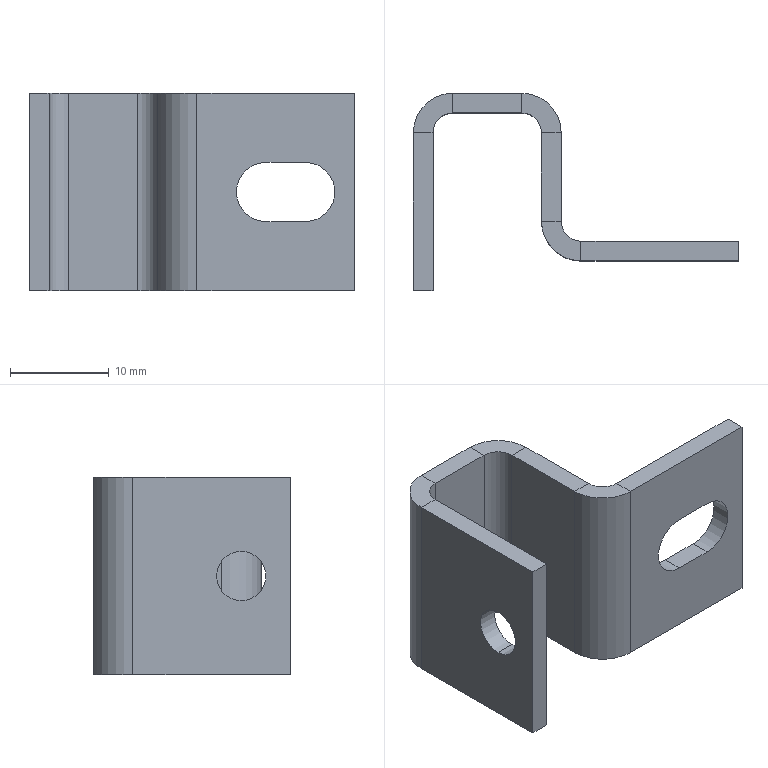Component | SolidWorks | Bracket(Item51)-1 | 1 solid | 36 faces | box 33 x 20 x 20 mm | volume 2342 mm3 | plane 26 | cylinder 10 | commonest cylinder face diameters 8 x3 4 x3 5 x2 6 x2 | material Plain Carbon Steel
STEP:
#1=COLOUR_RGB('',0.7922,0.8196,0.9333);
#2=FILL_AREA_STYLE_COLOUR('',#1);
#3=FILL_AREA_STYLE('',(#2));
#4=SURFACE_STYLE_FILL_AREA(#3);
#5=SURFACE_SIDE_STYLE('',(#4));
#6=SURFACE_STYLE_USAGE(.BOTH.,#5);
#7=PRESENTATION_STYLE_ASSIGNMENT((#6));
#8=CARTESIAN_POINT('',(-16.26,14.764,-4.528));
#9=VERTEX_POINT('',#8);
#10=CARTESIAN_POINT('',(-16.26,14.764,-4.331));
#11=VERTEX_POINT('',#10);
#12=CARTESIAN_POINT('',(-16.26,14.764,-4.429));
#13=DIRECTION('',(1.,-0.,0.));
#14=DIRECTION('',(0.,-1.,0.));
#15=AXIS2_PLACEMENT_3D('',#12,#13,#14);
#16=CIRCLE('',#15,0.09843);
#17=EDGE_CURVE('',#9,#11,#16,.T.);
#18=ORIENTED_EDGE('',*,*,#17,.T.);
#19=CARTESIAN_POINT('',(-16.339,14.764,-4.331));
#20=VERTEX_POINT('',#19);
#21=CARTESIAN_POINT('',(-16.339,14.764,-4.331));
#22=DIRECTION('',(-1.,0.,-0.));
#23=VECTOR('',#22,39.37);
#24=LINE('',#21,#23);
#25=EDGE_CURVE('',#11,#20,#24,.T.);
#26=ORIENTED_EDGE('',*,*,#25,.T.);
#27=CARTESIAN_POINT('',(-16.339,14.764,-4.528));
#28=VERTEX_POINT('',#27);
#29=CARTESIAN_POINT('',(-16.339,14.764,-4.429));
#30=DIRECTION('',(-1.,0.,-0.));
#31=DIRECTION('',(0.,0.,-1.));
#32=AXIS2_PLACEMENT_3D('',#29,#30,#31);
#33=CIRCLE('',#32,0.09843);
#34=EDGE_CURVE('',#20,#28,#33,.T.);
#35=ORIENTED_EDGE('',*,*,#34,.T.);
#36=CARTESIAN_POINT('',(-16.339,14.764,-4.528));
#37=DIRECTION('',(-1.,0.,-0.));
#38=VECTOR('',#37,39.37);
#39=LINE('',#36,#38);
#40=EDGE_CURVE('',#9,#28,#39,.T.);
#41=ORIENTED_EDGE('',*,*,#40,.F.);
#42=EDGE_LOOP('',(#18,#26,#35,#41));
#43=FACE_OUTER_BOUND('',#42,.T.);
#44=CARTESIAN_POINT('',(-16.339,14.764,-4.429));
#45=DIRECTION('',(-1.,0.,-0.));
#46=DIRECTION('',(0.,0.,-1.));
#47=AXIS2_PLACEMENT_3D('',#44,#45,#46);
#48=CYLINDRICAL_SURFACE('',#47,0.09843);
#49=ADVANCED_FACE('',(#43),#48,.F.);
#50=CARTESIAN_POINT('',(-16.339,15.197,-4.823));
#51=VERTEX_POINT('',#50);
#52=CARTESIAN_POINT('',(-16.26,15.197,-4.823));
#53=VERTEX_POINT('',#52);
#54=CARTESIAN_POINT('',(-16.339,15.197,-4.823));
#55=DIRECTION('',(1.,-0.,0.));
#56=VECTOR('',#55,39.37);
#57=LINE('',#54,#56);
#58=EDGE_CURVE('',#51,#53,#57,.T.);
#59=ORIENTED_EDGE('',*,*,#58,.F.);
#60=CARTESIAN_POINT('',(-16.181,15.354,-4.823));
#61=VERTEX_POINT('',#60);
#62=CARTESIAN_POINT('',(-16.181,15.197,-4.823));
#63=DIRECTION('',(0.,-0.,-1.));
#64=DIRECTION('',(-1.,0.,0.));
#65=AXIS2_PLACEMENT_3D('',#62,#63,#64);
#66=CIRCLE('',#65,0.1575);
#67=EDGE_CURVE('',#51,#61,#66,.T.);
#68=ORIENTED_EDGE('',*,*,#67,.T.);
#69=CARTESIAN_POINT('',(-16.181,15.276,-4.823));
#70=VERTEX_POINT('',#69);
#71=CARTESIAN_POINT('',(-16.181,15.276,-4.823));
#72=DIRECTION('',(0.,1.,-0.));
#73=VECTOR('',#72,39.37);
#74=LINE('',#71,#73);
#75=EDGE_CURVE('',#70,#61,#74,.T.);
#76=ORIENTED_EDGE('',*,*,#75,.F.);
#77=CARTESIAN_POINT('',(-16.181,15.197,-4.823));
#78=DIRECTION('',(0.,-0.,-1.));
#79=DIRECTION('',(1.,0.,0.));
#80=AXIS2_PLACEMENT_3D('',#77,#78,#79);
#81=CIRCLE('',#80,0.07874);
#82=EDGE_CURVE('',#53,#70,#81,.T.);
#83=ORIENTED_EDGE('',*,*,#82,.F.);
#84=EDGE_LOOP('',(#59,#68,#76,#83));
#85=FACE_OUTER_BOUND('',#84,.T.);
#86=CARTESIAN_POINT('',(-16.339,15.197,-4.823));
#87=DIRECTION('',(0.,-0.,-1.));
#88=DIRECTION('',(1.,-0.,0.));
#89=AXIS2_PLACEMENT_3D('',#86,#87,#88);
#90=PLANE('',#89);
#91=ADVANCED_FACE('',(#85),#90,.T.);
#92=CARTESIAN_POINT('',(-16.339,14.567,-4.823));
#93=VERTEX_POINT('',#92);
#94=CARTESIAN_POINT('',(-16.339,14.567,-4.823));
#95=DIRECTION('',(0.,1.,-0.));
#96=VECTOR('',#95,39.37);
#97=LINE('',#94,#96);
#98=EDGE_CURVE('',#93,#51,#97,.T.);
#99=ORIENTED_EDGE('',*,*,#98,.T.);
#100=ORIENTED_EDGE('',*,*,#58,.T.);
#101=CARTESIAN_POINT('',(-16.26,14.567,-4.823));
#102=VERTEX_POINT('',#101);
#103=CARTESIAN_POINT('',(-16.26,14.567,-4.823));
#104=DIRECTION('',(0.,1.,-0.));
#105=VECTOR('',#104,39.37);
#106=LINE('',#103,#105);
#107=EDGE_CURVE('',#102,#53,#106,.T.);
#108=ORIENTED_EDGE('',*,*,#107,.F.);
#109=CARTESIAN_POINT('',(-16.339,14.567,-4.823));
#110=DIRECTION('',(1.,-0.,0.));
#111=VECTOR('',#110,39.37);
#112=LINE('',#109,#111);
#113=EDGE_CURVE('',#93,#102,#112,.T.);
#114=ORIENTED_EDGE('',*,*,#113,.F.);
#115=EDGE_LOOP('',(#99,#100,#108,#114));
#116=FACE_OUTER_BOUND('',#115,.T.);
#117=CARTESIAN_POINT('',(-16.181,15.276,-4.823));
#118=DIRECTION('',(0.,-0.,-1.));
#119=DIRECTION('',(1.,-0.,0.));
#120=AXIS2_PLACEMENT_3D('',#117,#118,#119);
#121=PLANE('',#120);
#122=ADVANCED_FACE('',(#116),#121,.T.);
#123=CARTESIAN_POINT('',(-16.181,15.354,-4.035));
#124=VERTEX_POINT('',#123);
#125=CARTESIAN_POINT('',(-16.181,15.276,-4.035));
#126=VERTEX_POINT('',#125);
#127=CARTESIAN_POINT('',(-16.181,15.354,-4.035));
#128=DIRECTION('',(-0.,-1.,0.));
#129=VECTOR('',#128,39.37);
#130=LINE('',#127,#129);
#131=EDGE_CURVE('',#124,#126,#130,.T.);
#132=ORIENTED_EDGE('',*,*,#131,.F.);
#133=CARTESIAN_POINT('',(-16.339,15.197,-4.035));
#134=VERTEX_POINT('',#133);
#135=CARTESIAN_POINT('',(-16.181,15.197,-4.035));
#136=DIRECTION('',(0.,-0.,-1.));
#137=DIRECTION('',(-1.,0.,0.));
#138=AXIS2_PLACEMENT_3D('',#135,#136,#137);
#139=CIRCLE('',#138,0.1575);
#140=EDGE_CURVE('',#134,#124,#139,.T.);
#141=ORIENTED_EDGE('',*,*,#140,.F.);
#142=CARTESIAN_POINT('',(-16.26,15.197,-4.035));
#143=VERTEX_POINT('',#142);
#144=CARTESIAN_POINT('',(-16.26,15.197,-4.035));
#145=DIRECTION('',(-1.,0.,-0.));
#146=VECTOR('',#145,39.37);
#147=LINE('',#144,#146);
#148=EDGE_CURVE('',#143,#134,#147,.T.);
#149=ORIENTED_EDGE('',*,*,#148,.F.);
#150=CARTESIAN_POINT('',(-16.181,15.197,-4.035));
#151=DIRECTION('',(0.,-0.,-1.));
#152=DIRECTION('',(1.,0.,0.));
#153=AXIS2_PLACEMENT_3D('',#150,#151,#152);
#154=CIRCLE('',#153,0.07874);
#155=EDGE_CURVE('',#143,#126,#154,.T.);
#156=ORIENTED_EDGE('',*,*,#155,.T.);
#157=EDGE_LOOP('',(#132,#141,#149,#156));
#158=FACE_OUTER_BOUND('',#157,.T.);
#159=CARTESIAN_POINT('',(-16.181,15.354,-4.035));
#160=DIRECTION('',(-0.,0.,1.));
#161=DIRECTION('',(-1.,0.,-0.));
#162=AXIS2_PLACEMENT_3D('',#159,#160,#161);
#163=PLANE('',#162);
#164=ADVANCED_FACE('',(#158),#163,.T.);
#165=CARTESIAN_POINT('',(-15.906,15.354,-4.035));
#166=VERTEX_POINT('',#165);
#167=CARTESIAN_POINT('',(-16.339,15.354,-4.035));
#168=DIRECTION('',(1.,-0.,0.));
#169=VECTOR('',#168,39.37);
#170=LINE('',#167,#169);
#171=EDGE_CURVE('',#124,#166,#170,.T.);
#172=ORIENTED_EDGE('',*,*,#171,.F.);
#173=ORIENTED_EDGE('',*,*,#131,.T.);
#174=CARTESIAN_POINT('',(-15.906,15.276,-4.035));
#175=VERTEX_POINT('',#174);
#176=CARTESIAN_POINT('',(-16.339,15.276,-4.035));
#177=DIRECTION('',(1.,-0.,0.));
#178=VECTOR('',#177,39.37);
#179=LINE('',#176,#178);
#180=EDGE_CURVE('',#126,#175,#179,.T.);
#181=ORIENTED_EDGE('',*,*,#180,.T.);
#182=CARTESIAN_POINT('',(-15.906,15.276,-4.035));
#183=DIRECTION('',(-0.,1.,-0.));
#184=VECTOR('',#183,39.37);
#185=LINE('',#182,#184);
#186=EDGE_CURVE('',#175,#166,#185,.T.);
#187=ORIENTED_EDGE('',*,*,#186,.T.);
#188=EDGE_LOOP('',(#172,#173,#181,#187));
#189=FACE_OUTER_BOUND('',#188,.T.);
#190=CARTESIAN_POINT('',(-16.26,15.197,-4.035));
#191=DIRECTION('',(-0.,0.,1.));
#192=DIRECTION('',(-1.,0.,-0.));
#193=AXIS2_PLACEMENT_3D('',#190,#191,#192);
#194=PLANE('',#193);
#195=ADVANCED_FACE('',(#189),#194,.T.);
#196=CARTESIAN_POINT('',(-15.906,15.354,-4.823));
#197=VERTEX_POINT('',#196);
#198=CARTESIAN_POINT('',(-15.906,15.276,-4.823));
#199=VERTEX_POINT('',#198);
#200=CARTESIAN_POINT('',(-15.906,15.354,-4.823));
#201=DIRECTION('',(0.,-1.,0.));
#202=VECTOR('',#201,39.37);
#203=LINE('',#200,#202);
#204=EDGE_CURVE('',#197,#199,#203,.T.);
#205=ORIENTED_EDGE('',*,*,#204,.F.);
#206=CARTESIAN_POINT('',(-15.748,15.197,-4.823));
#207=VERTEX_POINT('',#206);
#208=CARTESIAN_POINT('',(-15.906,15.197,-4.823));
#209=DIRECTION('',(0.,-0.,-1.));
#210=DIRECTION('',(-1.,0.,0.));
#211=AXIS2_PLACEMENT_3D('',#208,#209,#210);
#212=CIRCLE('',#211,0.1575);
#213=EDGE_CURVE('',#197,#207,#212,.T.);
#214=ORIENTED_EDGE('',*,*,#213,.T.);
#215=CARTESIAN_POINT('',(-15.827,15.197,-4.823));
#216=VERTEX_POINT('',#215);
#217=CARTESIAN_POINT('',(-15.827,15.197,-4.823));
#218=DIRECTION('',(1.,-0.,0.));
#219=VECTOR('',#218,39.37);
#220=LINE('',#217,#219);
#221=EDGE_CURVE('',#216,#207,#220,.T.);
#222=ORIENTED_EDGE('',*,*,#221,.F.);
#223=CARTESIAN_POINT('',(-15.906,15.197,-4.823));
#224=DIRECTION('',(0.,-0.,-1.));
#225=DIRECTION('',(1.,0.,0.));
#226=AXIS2_PLACEMENT_3D('',#223,#224,#225);
#227=CIRCLE('',#226,0.07874);
#228=EDGE_CURVE('',#199,#216,#227,.T.);
#229=ORIENTED_EDGE('',*,*,#228,.F.);
#230=EDGE_LOOP('',(#205,#214,#222,#229));
#231=FACE_OUTER_BOUND('',#230,.T.);
#232=CARTESIAN_POINT('',(-15.906,15.354,-4.823));
#233=DIRECTION('',(0.,-0.,-1.));
#234=DIRECTION('',(1.,-0.,0.));
#235=AXIS2_PLACEMENT_3D('',#232,#233,#234);
#236=PLANE('',#235);
#237=ADVANCED_FACE('',(#231),#236,.T.);
#238=CARTESIAN_POINT('',(-16.339,15.354,-4.823));
#239=DIRECTION('',(1.,-0.,0.));
#240=VECTOR('',#239,39.37);
#241=LINE('',#238,#240);
#242=EDGE_CURVE('',#61,#197,#241,.T.);
#243=ORIENTED_EDGE('',*,*,#242,.T.);
#244=ORIENTED_EDGE('',*,*,#204,.T.);
#245=CARTESIAN_POINT('',(-16.339,15.276,-4.823));
#246=DIRECTION('',(1.,-0.,0.));
#247=VECTOR('',#246,39.37);
#248=LINE('',#245,#247);
#249=EDGE_CURVE('',#70,#199,#248,.T.);
#250=ORIENTED_EDGE('',*,*,#249,.F.);
#251=ORIENTED_EDGE('',*,*,#75,.T.);
#252=EDGE_LOOP('',(#243,#244,#250,#251));
#253=FACE_OUTER_BOUND('',#252,.T.);
#254=CARTESIAN_POINT('',(-15.827,15.197,-4.823));
#255=DIRECTION('',(0.,-0.,-1.));
#256=DIRECTION('',(1.,-0.,0.));
#257=AXIS2_PLACEMENT_3D('',#254,#255,#256);
#258=PLANE('',#257);
#259=ADVANCED_FACE('',(#253),#258,.T.);
#260=CARTESIAN_POINT('',(-15.748,15.197,-4.035));
#261=VERTEX_POINT('',#260);
#262=CARTESIAN_POINT('',(-15.827,15.197,-4.035));
#263=VERTEX_POINT('',#262);
#264=CARTESIAN_POINT('',(-15.748,15.197,-4.035));
#265=DIRECTION('',(-1.,0.,-0.));
#266=VECTOR('',#265,39.37);
#267=LINE('',#264,#266);
#268=EDGE_CURVE('',#261,#263,#267,.T.);
#269=ORIENTED_EDGE('',*,*,#268,.F.);
#270=CARTESIAN_POINT('',(-15.906,15.197,-4.035));
#271=DIRECTION('',(0.,-0.,-1.));
#272=DIRECTION('',(-1.,0.,0.));
#273=AXIS2_PLACEMENT_3D('',#270,#271,#272);
#274=CIRCLE('',#273,0.1575);
#275=EDGE_CURVE('',#166,#261,#274,.T.);
#276=ORIENTED_EDGE('',*,*,#275,.F.);
#277=ORIENTED_EDGE('',*,*,#186,.F.);
#278=CARTESIAN_POINT('',(-15.906,15.197,-4.035));
#279=DIRECTION('',(0.,-0.,-1.));
#280=DIRECTION('',(1.,0.,0.));
#281=AXIS2_PLACEMENT_3D('',#278,#279,#280);
#282=CIRCLE('',#281,0.07874);
#283=EDGE_CURVE('',#175,#263,#282,.T.);
#284=ORIENTED_EDGE('',*,*,#283,.T.);
#285=EDGE_LOOP('',(#269,#276,#277,#284));
#286=FACE_OUTER_BOUND('',#285,.T.);
#287=CARTESIAN_POINT('',(-15.748,15.197,-4.035));
#288=DIRECTION('',(-0.,0.,1.));
#289=DIRECTION('',(-1.,0.,-0.));
#290=AXIS2_PLACEMENT_3D('',#287,#288,#289);
#291=PLANE('',#290);
#292=ADVANCED_FACE('',(#286),#291,.T.);
#293=CARTESIAN_POINT('',(-15.748,14.843,-4.035));
#294=VERTEX_POINT('',#293);
#295=CARTESIAN_POINT('',(-15.748,15.354,-4.035));
#296=DIRECTION('',(0.,-1.,0.));
#297=VECTOR('',#296,39.37);
#298=LINE('',#295,#297);
#299=EDGE_CURVE('',#261,#294,#298,.T.);
#300=ORIENTED_EDGE('',*,*,#299,.F.);
#301=ORIENTED_EDGE('',*,*,#268,.T.);
#302=CARTESIAN_POINT('',(-15.827,14.843,-4.035));
#303=VERTEX_POINT('',#302);
#304=CARTESIAN_POINT('',(-15.827,15.354,-4.035));
#305=DIRECTION('',(0.,-1.,0.));
#306=VECTOR('',#305,39.37);
#307=LINE('',#304,#306);
#308=EDGE_CURVE('',#263,#303,#307,.T.);
#309=ORIENTED_EDGE('',*,*,#308,.T.);
#310=CARTESIAN_POINT('',(-15.827,14.843,-4.035));
#311=DIRECTION('',(1.,0.,0.));
#312=VECTOR('',#311,39.37);
#313=LINE('',#310,#312);
#314=EDGE_CURVE('',#303,#294,#313,.T.);
#315=ORIENTED_EDGE('',*,*,#314,.T.);
#316=EDGE_LOOP('',(#300,#301,#309,#315));
#317=FACE_OUTER_BOUND('',#316,.T.);
#318=CARTESIAN_POINT('',(-15.906,15.276,-4.035));
#319=DIRECTION('',(-0.,0.,1.));
#320=DIRECTION('',(-1.,0.,-0.));
#321=AXIS2_PLACEMENT_3D('',#318,#319,#320);
#322=PLANE('',#321);
#323=ADVANCED_FACE('',(#317),#322,.T.);
#324=CARTESIAN_POINT('',(-15.748,14.843,-4.823));
#325=VERTEX_POINT('',#324);
#326=CARTESIAN_POINT('',(-15.827,14.843,-4.823));
#327=VERTEX_POINT('',#326);
#328=CARTESIAN_POINT('',(-15.748,14.843,-4.823));
#329=DIRECTION('',(-1.,-0.,-0.));
#330=VECTOR('',#329,39.37);
#331=LINE('',#328,#330);
#332=EDGE_CURVE('',#325,#327,#331,.T.);
#333=ORIENTED_EDGE('',*,*,#332,.F.);
#334=CARTESIAN_POINT('',(-15.669,14.764,-4.823));
#335=VERTEX_POINT('',#334);
#336=CARTESIAN_POINT('',(-15.669,14.843,-4.823));
#337=DIRECTION('',(-0.,0.,1.));
#338=DIRECTION('',(1.,0.,0.));
#339=AXIS2_PLACEMENT_3D('',#336,#337,#338);
#340=CIRCLE('',#339,0.07874);
#341=EDGE_CURVE('',#325,#335,#340,.T.);
#342=ORIENTED_EDGE('',*,*,#341,.T.);
#343=CARTESIAN_POINT('',(-15.669,14.685,-4.823));
#344=VERTEX_POINT('',#343);
#345=CARTESIAN_POINT('',(-15.669,14.685,-4.823));
#346=DIRECTION('',(0.,1.,-0.));
#347=VECTOR('',#346,39.37);
#348=LINE('',#345,#347);
#349=EDGE_CURVE('',#344,#335,#348,.T.);
#350=ORIENTED_EDGE('',*,*,#349,.F.);
#351=CARTESIAN_POINT('',(-15.669,14.843,-4.823));
#352=DIRECTION('',(-0.,0.,1.));
#353=DIRECTION('',(1.,0.,0.));
#354=AXIS2_PLACEMENT_3D('',#351,#352,#353);
#355=CIRCLE('',#354,0.1575);
#356=EDGE_CURVE('',#327,#344,#355,.T.);
#357=ORIENTED_EDGE('',*,*,#356,.F.);
#358=EDGE_LOOP('',(#333,#342,#350,#357));
#359=FACE_OUTER_BOUND('',#358,.T.);
#360=CARTESIAN_POINT('',(-15.748,14.843,-4.823));
#361=DIRECTION('',(0.,-0.,-1.));
#362=DIRECTION('',(1.,-0.,0.));
#363=AXIS2_PLACEMENT_3D('',#360,#361,#362);
#364=PLANE('',#363);
#365=ADVANCED_FACE('',(#359),#364,.T.);
#366=CARTESIAN_POINT('',(-15.748,15.354,-4.823));
#367=DIRECTION('',(0.,-1.,0.));
#368=VECTOR('',#367,39.37);
#369=LINE('',#366,#368);
#370=EDGE_CURVE('',#207,#325,#369,.T.);
#371=ORIENTED_EDGE('',*,*,#370,.T.);
#372=ORIENTED_EDGE('',*,*,#332,.T.);
#373=CARTESIAN_POINT('',(-15.827,15.354,-4.823));
#374=DIRECTION('',(0.,-1.,0.));
#375=VECTOR('',#374,39.37);
#376=LINE('',#373,#375);
#377=EDGE_CURVE('',#216,#327,#376,.T.);
#378=ORIENTED_EDGE('',*,*,#377,.F.);
#379=ORIENTED_EDGE('',*,*,#221,.T.);
#380=EDGE_LOOP('',(#371,#372,#378,#379));
#381=FACE_OUTER_BOUND('',#380,.T.);
#382=CARTESIAN_POINT('',(-15.669,14.685,-4.823));
#383=DIRECTION('',(0.,-0.,-1.));
#384=DIRECTION('',(1.,-0.,0.));
#385=AXIS2_PLACEMENT_3D('',#382,#383,#384);
#386=PLANE('',#385);
#387=ADVANCED_FACE('',(#381),#386,.T.);
#388=CARTESIAN_POINT('',(-15.669,14.764,-4.035));
#389=VERTEX_POINT('',#388);
#390=CARTESIAN_POINT('',(-15.669,14.685,-4.035));
#391=VERTEX_POINT('',#390);
#392=CARTESIAN_POINT('',(-15.669,14.764,-4.035));
#393=DIRECTION('',(-0.,-1.,0.));
#394=VECTOR('',#393,39.37);
#395=LINE('',#392,#394);
#396=EDGE_CURVE('',#389,#391,#395,.T.);
#397=ORIENTED_EDGE('',*,*,#396,.F.);
#398=CARTESIAN_POINT('',(-15.669,14.843,-4.035));
#399=DIRECTION('',(-0.,0.,1.));
#400=DIRECTION('',(1.,0.,0.));
#401=AXIS2_PLACEMENT_3D('',#398,#399,#400);
#402=CIRCLE('',#401,0.07874);
#403=EDGE_CURVE('',#294,#389,#402,.T.);
#404=ORIENTED_EDGE('',*,*,#403,.F.);
#405=ORIENTED_EDGE('',*,*,#314,.F.);
#406=CARTESIAN_POINT('',(-15.669,14.843,-4.035));
#407=DIRECTION('',(-0.,0.,1.));
#408=DIRECTION('',(1.,0.,0.));
#409=AXIS2_PLACEMENT_3D('',#406,#407,#408);
#410=CIRCLE('',#409,0.1575);
#411=EDGE_CURVE('',#303,#391,#410,.T.);
#412=ORIENTED_EDGE('',*,*,#411,.T.);
#413=EDGE_LOOP('',(#397,#404,#405,#412));
#414=FACE_OUTER_BOUND('',#413,.T.);
#415=CARTESIAN_POINT('',(-15.669,14.764,-4.035));
#416=DIRECTION('',(-0.,0.,1.));
#417=DIRECTION('',(-1.,0.,-0.));
#418=AXIS2_PLACEMENT_3D('',#415,#416,#417);
#419=PLANE('',#418);
#420=ADVANCED_FACE('',(#414),#419,.T.);
#421=CARTESIAN_POINT('',(-15.039,14.764,-4.035));
#422=VERTEX_POINT('',#421);
#423=CARTESIAN_POINT('',(-15.748,14.764,-4.035));
#424=DIRECTION('',(1.,-0.,0.));
#425=VECTOR('',#424,39.37);
#426=LINE('',#423,#425);
#427=EDGE_CURVE('',#389,#422,#426,.T.);
#428=ORIENTED_EDGE('',*,*,#427,.F.);
#429=ORIENTED_EDGE('',*,*,#396,.T.);
#430=CARTESIAN_POINT('',(-15.039,14.685,-4.035));
#431=VERTEX_POINT('',#430);
#432=CARTESIAN_POINT('',(-15.748,14.685,-4.035));
#433=DIRECTION('',(1.,-0.,0.));
#434=VECTOR('',#433,39.37);
#435=LINE('',#432,#434);
#436=EDGE_CURVE('',#391,#431,#435,.T.);
#437=ORIENTED_EDGE('',*,*,#436,.T.);
#438=CARTESIAN_POINT('',(-15.039,14.685,-4.035));
#439=DIRECTION('',(0.,1.,-0.));
#440=VECTOR('',#439,39.37);
#441=LINE('',#438,#440);
#442=EDGE_CURVE('',#431,#422,#441,.T.);
#443=ORIENTED_EDGE('',*,*,#442,.T.);
#444=EDGE_LOOP('',(#428,#429,#437,#443));
#445=FACE_OUTER_BOUND('',#444,.T.);
#446=CARTESIAN_POINT('',(-15.827,14.843,-4.035));
#447=DIRECTION('',(-0.,0.,1.));
#448=DIRECTION('',(-1.,0.,-0.));
#449=AXIS2_PLACEMENT_3D('',#446,#447,#448);
#450=PLANE('',#449);
#451=ADVANCED_FACE('',(#445),#450,.T.);
#452=CARTESIAN_POINT('',(-15.236,14.764,-4.311));
#453=VERTEX_POINT('',#452);
#454=CARTESIAN_POINT('',(-15.394,14.764,-4.311));
#455=VERTEX_POINT('',#454);
#456=CARTESIAN_POINT('',(-15.394,14.764,-4.311));
#457=DIRECTION('',(-1.,0.,-0.));
#458=VECTOR('',#457,39.37);
#459=LINE('',#456,#458);
#460=EDGE_CURVE('',#453,#455,#459,.T.);
#461=ORIENTED_EDGE('',*,*,#460,.T.);
#462=CARTESIAN_POINT('',(-15.394,14.764,-4.547));
#463=VERTEX_POINT('',#462);
#464=CARTESIAN_POINT('',(-15.394,14.764,-4.429));
#465=DIRECTION('',(-0.,-1.,0.));
#466=DIRECTION('',(0.,0.,-1.));
#467=AXIS2_PLACEMENT_3D('',#464,#465,#466);
#468=CIRCLE('',#467,0.1181);
#469=EDGE_CURVE('',#455,#463,#468,.T.);
#470=ORIENTED_EDGE('',*,*,#469,.T.);
#471=CARTESIAN_POINT('',(-15.236,14.764,-4.547));
#472=VERTEX_POINT('',#471);
#473=CARTESIAN_POINT('',(-15.394,14.764,-4.547));
#474=DIRECTION('',(1.,-0.,0.));
#475=VECTOR('',#474,39.37);
#476=LINE('',#473,#475);
#477=EDGE_CURVE('',#463,#472,#476,.T.);
#478=ORIENTED_EDGE('',*,*,#477,.T.);
#479=CARTESIAN_POINT('',(-15.236,14.764,-4.429));
#480=DIRECTION('',(-0.,-1.,0.));
#481=DIRECTION('',(0.,0.,-1.));
#482=AXIS2_PLACEMENT_3D('',#479,#480,#481);
#483=CIRCLE('',#482,0.1181);
#484=EDGE_CURVE('',#472,#453,#483,.T.);
#485=ORIENTED_EDGE('',*,*,#484,.T.);
#486=EDGE_LOOP('',(#461,#470,#478,#485));
#487=FACE_BOUND('',#486,.T.);
#488=ORIENTED_EDGE('',*,*,#427,.T.);
#489=CARTESIAN_POINT('',(-15.039,14.764,-4.823));
#490=VERTEX_POINT('',#489);
#491=CARTESIAN_POINT('',(-15.039,14.764,-4.823));
#492=DIRECTION('',(-0.,0.,1.));
#493=VECTOR('',#492,39.37);
#494=LINE('',#491,#493);
#495=EDGE_CURVE('',#490,#422,#494,.T.);
#496=ORIENTED_EDGE('',*,*,#495,.F.);
#497=CARTESIAN_POINT('',(-15.748,14.764,-4.823));
#498=DIRECTION('',(1.,-0.,0.));
#499=VECTOR('',#498,39.37);
#500=LINE('',#497,#499);
#501=EDGE_CURVE('',#335,#490,#500,.T.);
#502=ORIENTED_EDGE('',*,*,#501,.F.);
#503=CARTESIAN_POINT('',(-15.669,14.764,-4.823));
#504=DIRECTION('',(-0.,0.,1.));
#505=VECTOR('',#504,39.37);
#506=LINE('',#503,#505);
#507=EDGE_CURVE('',#335,#389,#506,.T.);
#508=ORIENTED_EDGE('',*,*,#507,.T.);
#509=EDGE_LOOP('',(#488,#496,#502,#508));
#510=FACE_OUTER_BOUND('',#509,.T.);
#511=CARTESIAN_POINT('',(-15.748,14.764,-4.823));
#512=DIRECTION('',(-0.,-1.,0.));
#513=DIRECTION('',(0.,-0.,-1.));
#514=AXIS2_PLACEMENT_3D('',#511,#512,#513);
#515=PLANE('',#514);
#516=ADVANCED_FACE('',(#487,#510),#515,.F.);
#517=ORIENTED_EDGE('',*,*,#442,.F.);
#518=CARTESIAN_POINT('',(-15.039,14.685,-4.823));
#519=VERTEX_POINT('',#518);
#520=CARTESIAN_POINT('',(-15.039,14.685,-4.823));
#521=DIRECTION('',(-0.,0.,1.));
#522=VECTOR('',#521,39.37);
#523=LINE('',#520,#522);
#524=EDGE_CURVE('',#519,#431,#523,.T.);
#525=ORIENTED_EDGE('',*,*,#524,.F.);
#526=CARTESIAN_POINT('',(-15.039,14.685,-4.823));
#527=DIRECTION('',(0.,1.,-0.));
#528=VECTOR('',#527,39.37);
#529=LINE('',#526,#528);
#530=EDGE_CURVE('',#519,#490,#529,.T.);
#531=ORIENTED_EDGE('',*,*,#530,.T.);
#532=ORIENTED_EDGE('',*,*,#495,.T.);
#533=EDGE_LOOP('',(#517,#525,#531,#532));
#534=FACE_OUTER_BOUND('',#533,.T.);
#535=CARTESIAN_POINT('',(-15.039,14.685,-4.823));
#536=DIRECTION('',(1.,-0.,0.));
#537=DIRECTION('',(-0.,0.,1.));
#538=AXIS2_PLACEMENT_3D('',#535,#536,#537);
#539=PLANE('',#538);
#540=ADVANCED_FACE('',(#534),#539,.T.);
#541=CARTESIAN_POINT('',(-15.394,14.685,-4.311));
#542=VERTEX_POINT('',#541);
#543=CARTESIAN_POINT('',(-15.394,14.685,-4.547));
#544=VERTEX_POINT('',#543);
#545=CARTESIAN_POINT('',(-15.394,14.685,-4.429));
#546=DIRECTION('',(-0.,-1.,0.));
#547=DIRECTION('',(0.,0.,-1.));
#548=AXIS2_PLACEMENT_3D('',#545,#546,#547);
#549=CIRCLE('',#548,0.1181);
#550=EDGE_CURVE('',#542,#544,#549,.T.);
#551=ORIENTED_EDGE('',*,*,#550,.F.);
#552=CARTESIAN_POINT('',(-15.236,14.685,-4.311));
#553=VERTEX_POINT('',#552);
#554=CARTESIAN_POINT('',(-15.394,14.685,-4.311));
#555=DIRECTION('',(-1.,0.,-0.));
#556=VECTOR('',#555,39.37);
#557=LINE('',#554,#556);
#558=EDGE_CURVE('',#553,#542,#557,.T.);
#559=ORIENTED_EDGE('',*,*,#558,.F.);
#560=CARTESIAN_POINT('',(-15.236,14.685,-4.547));
#561=VERTEX_POINT('',#560);
#562=CARTESIAN_POINT('',(-15.236,14.685,-4.429));
#563=DIRECTION('',(-0.,-1.,0.));
#564=DIRECTION('',(0.,0.,-1.));
#565=AXIS2_PLACEMENT_3D('',#562,#563,#564);
#566=CIRCLE('',#565,0.1181);
#567=EDGE_CURVE('',#561,#553,#566,.T.);
#568=ORIENTED_EDGE('',*,*,#567,.F.);
#569=CARTESIAN_POINT('',(-15.394,14.685,-4.547));
#570=DIRECTION('',(1.,-0.,0.));
#571=VECTOR('',#570,39.37);
#572=LINE('',#569,#571);
#573=EDGE_CURVE('',#544,#561,#572,.T.);
#574=ORIENTED_EDGE('',*,*,#573,.F.);
#575=EDGE_LOOP('',(#551,#559,#568,#574));
#576=FACE_BOUND('',#575,.T.);
#577=ORIENTED_EDGE('',*,*,#436,.F.);
#578=CARTESIAN_POINT('',(-15.669,14.685,-4.823));
#579=DIRECTION('',(-0.,0.,1.));
#580=VECTOR('',#579,39.37);
#581=LINE('',#578,#580);
#582=EDGE_CURVE('',#344,#391,#581,.T.);
#583=ORIENTED_EDGE('',*,*,#582,.F.);
#584=CARTESIAN_POINT('',(-15.748,14.685,-4.823));
#585=DIRECTION('',(1.,-0.,0.));
#586=VECTOR('',#585,39.37);
#587=LINE('',#584,#586);
#588=EDGE_CURVE('',#344,#519,#587,.T.);
#589=ORIENTED_EDGE('',*,*,#588,.T.);
#590=ORIENTED_EDGE('',*,*,#524,.T.);
#591=EDGE_LOOP('',(#577,#583,#589,#590));
#592=FACE_OUTER_BOUND('',#591,.T.);
#593=CARTESIAN_POINT('',(-15.748,14.685,-4.823));
#594=DIRECTION('',(-0.,-1.,0.));
#595=DIRECTION('',(0.,-0.,-1.));
#596=AXIS2_PLACEMENT_3D('',#593,#594,#595);
#597=PLANE('',#596);
#598=ADVANCED_FACE('',(#576,#592),#597,.T.);
#599=ORIENTED_EDGE('',*,*,#411,.F.);
#600=CARTESIAN_POINT('',(-15.827,14.843,-4.823));
#601=DIRECTION('',(-0.,0.,1.));
#602=VECTOR('',#601,39.37);
#603=LINE('',#600,#602);
#604=EDGE_CURVE('',#327,#303,#603,.T.);
#605=ORIENTED_EDGE('',*,*,#604,.F.);
#606=ORIENTED_EDGE('',*,*,#356,.T.);
#607=ORIENTED_EDGE('',*,*,#582,.T.);
#608=EDGE_LOOP('',(#599,#605,#606,#607));
#609=FACE_OUTER_BOUND('',#608,.T.);
#610=CARTESIAN_POINT('',(-15.669,14.843,-4.823));
#611=DIRECTION('',(-0.,0.,1.));
#612=DIRECTION('',(-1.,0.,0.));
#613=AXIS2_PLACEMENT_3D('',#610,#611,#612);
#614=CYLINDRICAL_SURFACE('',#613,0.1575);
#615=ADVANCED_FACE('',(#609),#614,.T.);
#616=ORIENTED_EDGE('',*,*,#308,.F.);
#617=CARTESIAN_POINT('',(-15.827,15.197,-4.823));
#618=DIRECTION('',(-0.,0.,1.));
#619=VECTOR('',#618,39.37);
#620=LINE('',#617,#619);
#621=EDGE_CURVE('',#216,#263,#620,.T.);
#622=ORIENTED_EDGE('',*,*,#621,.F.);
#623=ORIENTED_EDGE('',*,*,#377,.T.);
#624=ORIENTED_EDGE('',*,*,#604,.T.);
#625=EDGE_LOOP('',(#616,#622,#623,#624));
#626=FACE_OUTER_BOUND('',#625,.T.);
#627=CARTESIAN_POINT('',(-15.827,15.354,-4.823));
#628=DIRECTION('',(-1.,-0.,-0.));
#629=DIRECTION('',(-0.,1.,-0.));
#630=AXIS2_PLACEMENT_3D('',#627,#628,#629);
#631=PLANE('',#630);
#632=ADVANCED_FACE('',(#626),#631,.T.);
#633=ORIENTED_EDGE('',*,*,#283,.F.);
#634=CARTESIAN_POINT('',(-15.906,15.276,-4.823));
#635=DIRECTION('',(-0.,0.,1.));
#636=VECTOR('',#635,39.37);
#637=LINE('',#634,#636);
#638=EDGE_CURVE('',#199,#175,#637,.T.);
#639=ORIENTED_EDGE('',*,*,#638,.F.);
#640=ORIENTED_EDGE('',*,*,#228,.T.);
#641=ORIENTED_EDGE('',*,*,#621,.T.);
#642=EDGE_LOOP('',(#633,#639,#640,#641));
#643=FACE_OUTER_BOUND('',#642,.T.);
#644=CARTESIAN_POINT('',(-15.906,15.197,-4.823));
#645=DIRECTION('',(-0.,0.,1.));
#646=DIRECTION('',(-1.,0.,0.));
#647=AXIS2_PLACEMENT_3D('',#644,#645,#646);
#648=CYLINDRICAL_SURFACE('',#647,0.07874);
#649=ADVANCED_FACE('',(#643),#648,.F.);
#650=ORIENTED_EDGE('',*,*,#180,.F.);
#651=CARTESIAN_POINT('',(-16.181,15.276,-4.823));
#652=DIRECTION('',(-0.,0.,1.));
#653=VECTOR('',#652,39.37);
#654=LINE('',#651,#653);
#655=EDGE_CURVE('',#70,#126,#654,.T.);
#656=ORIENTED_EDGE('',*,*,#655,.F.);
#657=ORIENTED_EDGE('',*,*,#249,.T.);
#658=ORIENTED_EDGE('',*,*,#638,.T.);
#659=EDGE_LOOP('',(#650,#656,#657,#658));
#660=FACE_OUTER_BOUND('',#659,.T.);
#661=CARTESIAN_POINT('',(-16.339,15.276,-4.823));
#662=DIRECTION('',(-0.,-1.,0.));
#663=DIRECTION('',(0.,-0.,-1.));
#664=AXIS2_PLACEMENT_3D('',#661,#662,#663);
#665=PLANE('',#664);
#666=ADVANCED_FACE('',(#660),#665,.T.);
#667=ORIENTED_EDGE('',*,*,#155,.F.);
#668=CARTESIAN_POINT('',(-16.26,15.197,-4.823));
#669=DIRECTION('',(-0.,0.,1.));
#670=VECTOR('',#669,39.37);
#671=LINE('',#668,#670);
#672=EDGE_CURVE('',#53,#143,#671,.T.);
#673=ORIENTED_EDGE('',*,*,#672,.F.);
#674=ORIENTED_EDGE('',*,*,#82,.T.);
#675=ORIENTED_EDGE('',*,*,#655,.T.);
#676=EDGE_LOOP('',(#667,#673,#674,#675));
#677=FACE_OUTER_BOUND('',#676,.T.);
#678=CARTESIAN_POINT('',(-16.181,15.197,-4.823));
#679=DIRECTION('',(-0.,0.,1.));
#680=DIRECTION('',(-1.,0.,0.));
#681=AXIS2_PLACEMENT_3D('',#678,#679,#680);
#682=CYLINDRICAL_SURFACE('',#681,0.07874);
#683=ADVANCED_FACE('',(#677),#682,.F.);
#684=ORIENTED_EDGE('',*,*,#17,.F.);
#685=CARTESIAN_POINT('',(-16.26,14.764,-4.429));
#686=DIRECTION('',(1.,-0.,0.));
#687=DIRECTION('',(0.,-1.,0.));
#688=AXIS2_PLACEMENT_3D('',#685,#686,#687);
#689=CIRCLE('',#688,0.09843);
#690=EDGE_CURVE('',#11,#9,#689,.T.);
#691=ORIENTED_EDGE('',*,*,#690,.F.);
#692=EDGE_LOOP('',(#684,#691));
#693=FACE_BOUND('',#692,.T.);
#694=CARTESIAN_POINT('',(-16.26,14.567,-4.035));
#695=VERTEX_POINT('',#694);
#696=CARTESIAN_POINT('',(-16.26,14.567,-4.035));
#697=DIRECTION('',(0.,1.,-0.));
#698=VECTOR('',#697,39.37);
#699=LINE('',#696,#698);
#700=EDGE_CURVE('',#695,#143,#699,.T.);
#701=ORIENTED_EDGE('',*,*,#700,.F.);
#702=CARTESIAN_POINT('',(-16.26,14.567,-4.823));
#703=DIRECTION('',(-0.,0.,1.));
#704=VECTOR('',#703,39.37);
#705=LINE('',#702,#704);
#706=EDGE_CURVE('',#102,#695,#705,.T.);
#707=ORIENTED_EDGE('',*,*,#706,.F.);
#708=ORIENTED_EDGE('',*,*,#107,.T.);
#709=ORIENTED_EDGE('',*,*,#672,.T.);
#710=EDGE_LOOP('',(#701,#707,#708,#709));
#711=FACE_OUTER_BOUND('',#710,.T.);
#712=CARTESIAN_POINT('',(-16.26,14.567,-4.823));
#713=DIRECTION('',(1.,-0.,0.));
#714=DIRECTION('',(-0.,-1.,0.));
#715=AXIS2_PLACEMENT_3D('',#712,#713,#714);
#716=PLANE('',#715);
#717=ADVANCED_FACE('',(#693,#711),#716,.T.);
#718=CARTESIAN_POINT('',(-16.339,14.567,-4.035));
#719=VERTEX_POINT('',#718);
#720=CARTESIAN_POINT('',(-16.339,14.567,-4.035));
#721=DIRECTION('',(1.,-0.,0.));
#722=VECTOR('',#721,39.37);
#723=LINE('',#720,#722);
#724=EDGE_CURVE('',#719,#695,#723,.T.);
#725=ORIENTED_EDGE('',*,*,#724,.F.);
#726=CARTESIAN_POINT('',(-16.339,14.567,-4.823));
#727=DIRECTION('',(-0.,0.,1.));
#728=VECTOR('',#727,39.37);
#729=LINE('',#726,#728);
#730=EDGE_CURVE('',#93,#719,#729,.T.);
#731=ORIENTED_EDGE('',*,*,#730,.F.);
#732=ORIENTED_EDGE('',*,*,#113,.T.);
#733=ORIENTED_EDGE('',*,*,#706,.T.);
#734=EDGE_LOOP('',(#725,#731,#732,#733));
#735=FACE_OUTER_BOUND('',#734,.T.);
#736=CARTESIAN_POINT('',(-16.339,14.567,-4.823));
#737=DIRECTION('',(-0.,-1.,0.));
#738=DIRECTION('',(-1.,0.,-0.));
#739=AXIS2_PLACEMENT_3D('',#736,#737,#738);
#740=PLANE('',#739);
#741=ADVANCED_FACE('',(#735),#740,.T.);
#742=CARTESIAN_POINT('',(-16.339,14.764,-4.429));
#743=DIRECTION('',(-1.,0.,-0.));
#744=DIRECTION('',(0.,0.,-1.));
#745=AXIS2_PLACEMENT_3D('',#742,#743,#744);
#746=CIRCLE('',#745,0.09843);
#747=EDGE_CURVE('',#28,#20,#746,.T.);
#748=ORIENTED_EDGE('',*,*,#747,.F.);
#749=ORIENTED_EDGE('',*,*,#34,.F.);
#750=EDGE_LOOP('',(#748,#749));
#751=FACE_BOUND('',#750,.T.);
#752=CARTESIAN_POINT('',(-16.339,14.567,-4.035));
#753=DIRECTION('',(0.,1.,-0.));
#754=VECTOR('',#753,39.37);
#755=LINE('',#752,#754);
#756=EDGE_CURVE('',#719,#134,#755,.T.);
#757=ORIENTED_EDGE('',*,*,#756,.T.);
#758=CARTESIAN_POINT('',(-16.339,15.197,-4.823));
#759=DIRECTION('',(-0.,0.,1.));
#760=VECTOR('',#759,39.37);
#761=LINE('',#758,#760);
#762=EDGE_CURVE('',#51,#134,#761,.T.);
#763=ORIENTED_EDGE('',*,*,#762,.F.);
#764=ORIENTED_EDGE('',*,*,#98,.F.);
#765=ORIENTED_EDGE('',*,*,#730,.T.);
#766=EDGE_LOOP('',(#757,#763,#764,#765));
#767=FACE_OUTER_BOUND('',#766,.T.);
#768=CARTESIAN_POINT('',(-16.339,14.567,-4.823));
#769=DIRECTION('',(1.,-0.,0.));
#770=DIRECTION('',(-0.,-1.,0.));
#771=AXIS2_PLACEMENT_3D('',#768,#769,#770);
#772=PLANE('',#771);
#773=ADVANCED_FACE('',(#751,#767),#772,.F.);
#774=ORIENTED_EDGE('',*,*,#140,.T.);
#775=CARTESIAN_POINT('',(-16.181,15.354,-4.823));
#776=DIRECTION('',(-0.,0.,1.));
#777=VECTOR('',#776,39.37);
#778=LINE('',#775,#777);
#779=EDGE_CURVE('',#61,#124,#778,.T.);
#780=ORIENTED_EDGE('',*,*,#779,.F.);
#781=ORIENTED_EDGE('',*,*,#67,.F.);
#782=ORIENTED_EDGE('',*,*,#762,.T.);
#783=EDGE_LOOP('',(#774,#780,#781,#782));
#784=FACE_OUTER_BOUND('',#783,.T.);
#785=CARTESIAN_POINT('',(-16.181,15.197,-4.823));
#786=DIRECTION('',(-0.,0.,1.));
#787=DIRECTION('',(-1.,0.,0.));
#788=AXIS2_PLACEMENT_3D('',#785,#786,#787);
#789=CYLINDRICAL_SURFACE('',#788,0.1575);
#790=ADVANCED_FACE('',(#784),#789,.T.);
#791=ORIENTED_EDGE('',*,*,#171,.T.);
#792=CARTESIAN_POINT('',(-15.906,15.354,-4.823));
#793=DIRECTION('',(-0.,0.,1.));
#794=VECTOR('',#793,39.37);
#795=LINE('',#792,#794);
#796=EDGE_CURVE('',#197,#166,#795,.T.);
#797=ORIENTED_EDGE('',*,*,#796,.F.);
#798=ORIENTED_EDGE('',*,*,#242,.F.);
#799=ORIENTED_EDGE('',*,*,#779,.T.);
#800=EDGE_LOOP('',(#791,#797,#798,#799));
#801=FACE_OUTER_BOUND('',#800,.T.);
#802=CARTESIAN_POINT('',(-16.339,15.354,-4.823));
#803=DIRECTION('',(-0.,-1.,0.));
#804=DIRECTION('',(0.,-0.,-1.));
#805=AXIS2_PLACEMENT_3D('',#802,#803,#804);
#806=PLANE('',#805);
#807=ADVANCED_FACE('',(#801),#806,.F.);
#808=ORIENTED_EDGE('',*,*,#275,.T.);
#809=CARTESIAN_POINT('',(-15.748,15.197,-4.823));
#810=DIRECTION('',(-0.,0.,1.));
#811=VECTOR('',#810,39.37);
#812=LINE('',#809,#811);
#813=EDGE_CURVE('',#207,#261,#812,.T.);
#814=ORIENTED_EDGE('',*,*,#813,.F.);
#815=ORIENTED_EDGE('',*,*,#213,.F.);
#816=ORIENTED_EDGE('',*,*,#796,.T.);
#817=EDGE_LOOP('',(#808,#814,#815,#816));
#818=FACE_OUTER_BOUND('',#817,.T.);
#819=CARTESIAN_POINT('',(-15.906,15.197,-4.823));
#820=DIRECTION('',(-0.,0.,1.));
#821=DIRECTION('',(-1.,0.,0.));
#822=AXIS2_PLACEMENT_3D('',#819,#820,#821);
#823=CYLINDRICAL_SURFACE('',#822,0.1575);
#824=ADVANCED_FACE('',(#818),#823,.T.);
#825=ORIENTED_EDGE('',*,*,#299,.T.);
#826=CARTESIAN_POINT('',(-15.748,14.843,-4.823));
#827=DIRECTION('',(-0.,0.,1.));
#828=VECTOR('',#827,39.37);
#829=LINE('',#826,#828);
#830=EDGE_CURVE('',#325,#294,#829,.T.);
#831=ORIENTED_EDGE('',*,*,#830,.F.);
#832=ORIENTED_EDGE('',*,*,#370,.F.);
#833=ORIENTED_EDGE('',*,*,#813,.T.);
#834=EDGE_LOOP('',(#825,#831,#832,#833));
#835=FACE_OUTER_BOUND('',#834,.T.);
#836=CARTESIAN_POINT('',(-15.748,15.354,-4.823));
#837=DIRECTION('',(-1.,-0.,-0.));
#838=DIRECTION('',(-0.,1.,-0.));
#839=AXIS2_PLACEMENT_3D('',#836,#837,#838);
#840=PLANE('',#839);
#841=ADVANCED_FACE('',(#835),#840,.F.);
#842=ORIENTED_EDGE('',*,*,#403,.T.);
#843=ORIENTED_EDGE('',*,*,#507,.F.);
#844=ORIENTED_EDGE('',*,*,#341,.F.);
#845=ORIENTED_EDGE('',*,*,#830,.T.);
#846=EDGE_LOOP('',(#842,#843,#844,#845));
#847=FACE_OUTER_BOUND('',#846,.T.);
#848=CARTESIAN_POINT('',(-15.669,14.843,-4.823));
#849=DIRECTION('',(-0.,0.,1.));
#850=DIRECTION('',(-1.,0.,0.));
#851=AXIS2_PLACEMENT_3D('',#848,#849,#850);
#852=CYLINDRICAL_SURFACE('',#851,0.07874);
#853=ADVANCED_FACE('',(#847),#852,.F.);
#854=ORIENTED_EDGE('',*,*,#501,.T.);
#855=ORIENTED_EDGE('',*,*,#530,.F.);
#856=ORIENTED_EDGE('',*,*,#588,.F.);
#857=ORIENTED_EDGE('',*,*,#349,.T.);
#858=EDGE_LOOP('',(#854,#855,#856,#857));
#859=FACE_OUTER_BOUND('',#858,.T.);
#860=CARTESIAN_POINT('',(-15.669,14.843,-4.823));
#861=DIRECTION('',(0.,-0.,-1.));
#862=DIRECTION('',(1.,-0.,0.));
#863=AXIS2_PLACEMENT_3D('',#860,#861,#862);
#864=PLANE('',#863);
#865=ADVANCED_FACE('',(#859),#864,.T.);
#866=ORIENTED_EDGE('',*,*,#700,.T.);
#867=ORIENTED_EDGE('',*,*,#148,.T.);
#868=ORIENTED_EDGE('',*,*,#756,.F.);
#869=ORIENTED_EDGE('',*,*,#724,.T.);
#870=EDGE_LOOP('',(#866,#867,#868,#869));
#871=FACE_OUTER_BOUND('',#870,.T.);
#872=CARTESIAN_POINT('',(-15.669,14.843,-4.035));
#873=DIRECTION('',(0.,-0.,-1.));
#874=DIRECTION('',(1.,-0.,0.));
#875=AXIS2_PLACEMENT_3D('',#872,#873,#874);
#876=PLANE('',#875);
#877=ADVANCED_FACE('',(#871),#876,.F.);
#878=ORIENTED_EDGE('',*,*,#25,.F.);
#879=ORIENTED_EDGE('',*,*,#690,.T.);
#880=ORIENTED_EDGE('',*,*,#40,.T.);
#881=ORIENTED_EDGE('',*,*,#747,.T.);
#882=EDGE_LOOP('',(#878,#879,#880,#881));
#883=FACE_OUTER_BOUND('',#882,.T.);
#884=CARTESIAN_POINT('',(-16.339,14.764,-4.429));
#885=DIRECTION('',(-1.,0.,-0.));
#886=DIRECTION('',(0.,0.,-1.));
#887=AXIS2_PLACEMENT_3D('',#884,#885,#886);
#888=CYLINDRICAL_SURFACE('',#887,0.09843);
#889=ADVANCED_FACE('',(#883),#888,.F.);
#890=ORIENTED_EDGE('',*,*,#550,.T.);
#891=CARTESIAN_POINT('',(-15.394,14.764,-4.547));
#892=DIRECTION('',(-0.,-1.,0.));
#893=VECTOR('',#892,39.37);
#894=LINE('',#891,#893);
#895=EDGE_CURVE('',#463,#544,#894,.T.);
#896=ORIENTED_EDGE('',*,*,#895,.F.);
#897=ORIENTED_EDGE('',*,*,#469,.F.);
#898=CARTESIAN_POINT('',(-15.394,14.764,-4.311));
#899=DIRECTION('',(-0.,-1.,0.));
#900=VECTOR('',#899,39.37);
#901=LINE('',#898,#900);
#902=EDGE_CURVE('',#455,#542,#901,.T.);
#903=ORIENTED_EDGE('',*,*,#902,.T.);
#904=EDGE_LOOP('',(#890,#896,#897,#903));
#905=FACE_OUTER_BOUND('',#904,.T.);
#906=CARTESIAN_POINT('',(-15.394,14.764,-4.429));
#907=DIRECTION('',(-0.,-1.,0.));
#908=DIRECTION('',(0.,0.,-1.));
#909=AXIS2_PLACEMENT_3D('',#906,#907,#908);
#910=CYLINDRICAL_SURFACE('',#909,0.1181);
#911=ADVANCED_FACE('',(#905),#910,.F.);
#912=ORIENTED_EDGE('',*,*,#558,.T.);
#913=ORIENTED_EDGE('',*,*,#902,.F.);
#914=ORIENTED_EDGE('',*,*,#460,.F.);
#915=CARTESIAN_POINT('',(-15.236,14.764,-4.311));
#916=DIRECTION('',(-0.,-1.,0.));
#917=VECTOR('',#916,39.37);
#918=LINE('',#915,#917);
#919=EDGE_CURVE('',#453,#553,#918,.T.);
#920=ORIENTED_EDGE('',*,*,#919,.T.);
#921=EDGE_LOOP('',(#912,#913,#914,#920));
#922=FACE_OUTER_BOUND('',#921,.T.);
#923=CARTESIAN_POINT('',(-15.394,14.764,-4.311));
#924=DIRECTION('',(-0.,0.,1.));
#925=DIRECTION('',(-1.,0.,-0.));
#926=AXIS2_PLACEMENT_3D('',#923,#924,#925);
#927=PLANE('',#926);
#928=ADVANCED_FACE('',(#922),#927,.F.);
#929=ORIENTED_EDGE('',*,*,#567,.T.);
#930=ORIENTED_EDGE('',*,*,#919,.F.);
#931=ORIENTED_EDGE('',*,*,#484,.F.);
#932=CARTESIAN_POINT('',(-15.236,14.764,-4.547));
#933=DIRECTION('',(-0.,-1.,0.));
#934=VECTOR('',#933,39.37);
#935=LINE('',#932,#934);
#936=EDGE_CURVE('',#472,#561,#935,.T.);
#937=ORIENTED_EDGE('',*,*,#936,.T.);
#938=EDGE_LOOP('',(#929,#930,#931,#937));
#939=FACE_OUTER_BOUND('',#938,.T.);
#940=CARTESIAN_POINT('',(-15.236,14.764,-4.429));
#941=DIRECTION('',(-0.,-1.,0.));
#942=DIRECTION('',(0.,0.,-1.));
#943=AXIS2_PLACEMENT_3D('',#940,#941,#942);
#944=CYLINDRICAL_SURFACE('',#943,0.1181);
#945=ADVANCED_FACE('',(#939),#944,.F.);
#946=ORIENTED_EDGE('',*,*,#573,.T.);
#947=ORIENTED_EDGE('',*,*,#936,.F.);
#948=ORIENTED_EDGE('',*,*,#477,.F.);
#949=ORIENTED_EDGE('',*,*,#895,.T.);
#950=EDGE_LOOP('',(#946,#947,#948,#949));
#951=FACE_OUTER_BOUND('',#950,.T.);
#952=CARTESIAN_POINT('',(-15.394,14.764,-4.547));
#953=DIRECTION('',(0.,-0.,-1.));
#954=DIRECTION('',(1.,-0.,0.));
#955=AXIS2_PLACEMENT_3D('',#952,#953,#954);
#956=PLANE('',#955);
#957=ADVANCED_FACE('',(#951),#956,.F.);
#958=CLOSED_SHELL('',(#49,#91,#122,#164,#195,#237,#259,#292,#323,#365,#387,#420,#451,#516,#540,#598,#615,#632,#649,#666,#683,#717,#741,#773,#790,#807,#824,#841,#853,#865,#877,#889,#911,#928,#945,#957));
#959=MANIFOLD_SOLID_BREP('',#958);
#960=STYLED_ITEM('',(#7),#959);
#961=(LENGTH_UNIT()NAMED_UNIT(*)SI_UNIT($,.METRE.));
#962=LENGTH_MEASURE_WITH_UNIT(LENGTH_MEASURE(0.0254),#961);
#963=DIMENSIONAL_EXPONENTS(1.,0.,0.,0.,0.,0.,0.);
#964=(CONVERSION_BASED_UNIT('',#962)LENGTH_UNIT()NAMED_UNIT(#963));
#965=UNCERTAINTY_MEASURE_WITH_UNIT(LENGTH_MEASURE(0.00001),#964,'','');
#966=(NAMED_UNIT(*)PLANE_ANGLE_UNIT()SI_UNIT($,.RADIAN.));
#967=(NAMED_UNIT(*)SI_UNIT($,.STERADIAN.)SOLID_ANGLE_UNIT());
#968=(GEOMETRIC_REPRESENTATION_CONTEXT(3)GLOBAL_UNCERTAINTY_ASSIGNED_CONTEXT((#965))GLOBAL_UNIT_ASSIGNED_CONTEXT((#964,#966,#967))REPRESENTATION_CONTEXT('',''));
#969=MECHANICAL_DESIGN_GEOMETRIC_PRESENTATION_REPRESENTATION('',(#960),#968);
#970=CARTESIAN_POINT('',(0.,0.,0.));
#971=DIRECTION('',(0.,0.,1.));
#972=DIRECTION('',(1.,0.,0.));
#973=AXIS2_PLACEMENT_3D('',#970,#971,#972);
#974=(LENGTH_UNIT()NAMED_UNIT(*)SI_UNIT($,.METRE.));
#975=LENGTH_MEASURE_WITH_UNIT(LENGTH_MEASURE(0.0254),#974);
#976=DIMENSIONAL_EXPONENTS(1.,0.,0.,0.,0.,0.,0.);
#977=(CONVERSION_BASED_UNIT('',#975)LENGTH_UNIT()NAMED_UNIT(#976));
#978=UNCERTAINTY_MEASURE_WITH_UNIT(LENGTH_MEASURE(0.00001),#977,'','');
#979=(NAMED_UNIT(*)PLANE_ANGLE_UNIT()SI_UNIT($,.RADIAN.));
#980=(NAMED_UNIT(*)SI_UNIT($,.STERADIAN.)SOLID_ANGLE_UNIT());
#981=(GEOMETRIC_REPRESENTATION_CONTEXT(3)GLOBAL_UNCERTAINTY_ASSIGNED_CONTEXT((#978))GLOBAL_UNIT_ASSIGNED_CONTEXT((#977,#979,#980))REPRESENTATION_CONTEXT('',''));
#982=ADVANCED_BREP_SHAPE_REPRESENTATION('',(#959,#973),#981);
#983=PRESENTATION_LAYER_ASSIGNMENT('','',(#960));